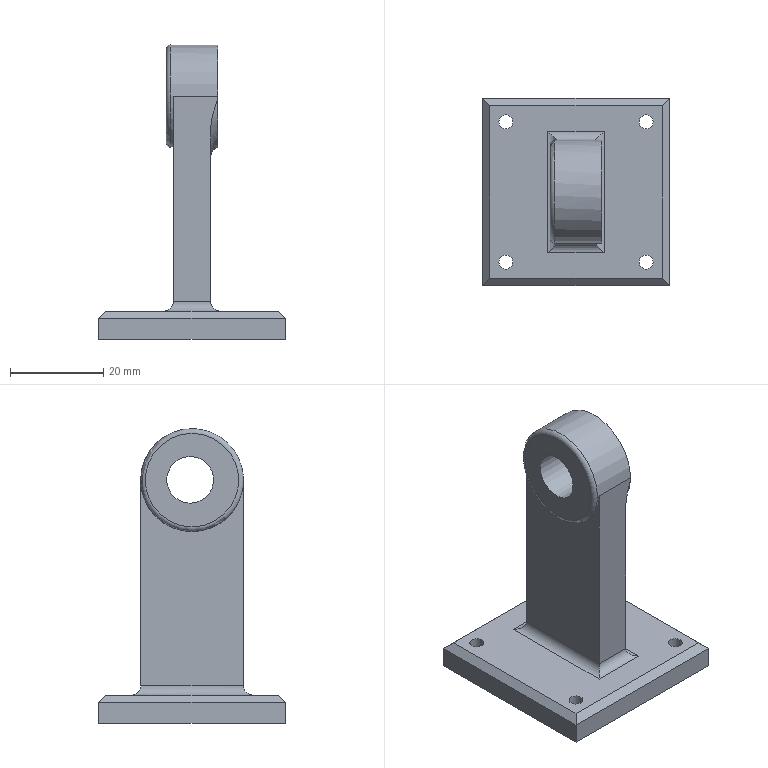Component | NX | ASSY_PRAC_PART_8 | 1 solid | 30 faces | volume 19017 mm3 | plane 16 | cylinder 11 | torus 2 | cone 1 | commonest cylinder face diameters 4 x4 3 x4 22 x1 14 x1 10 x1